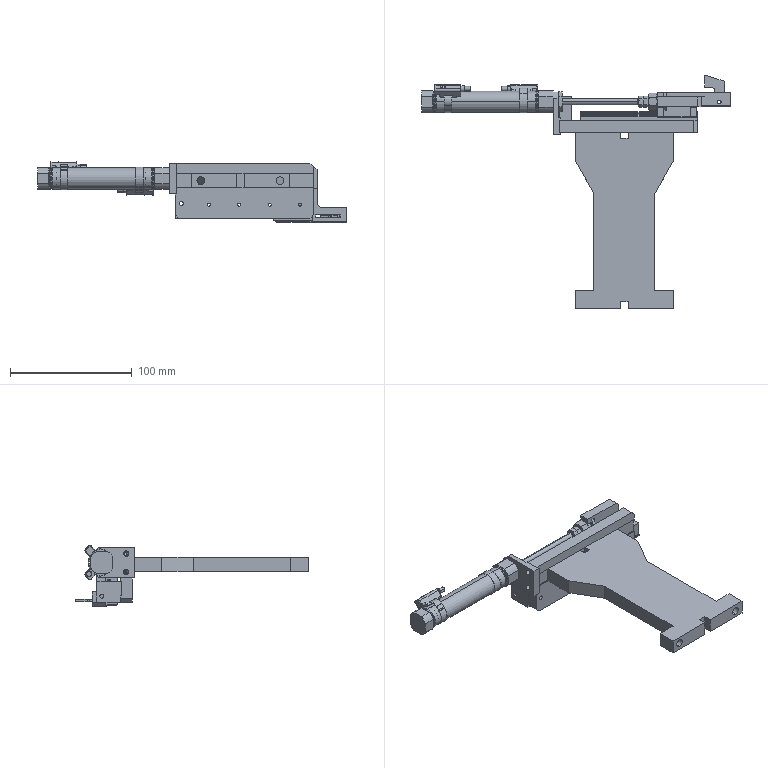Assembly | SolidWorks | mm | 16 component files | 16 solids | 740 faces | box 253.5 x 192.15 x 49.83 mm | volume 206829 mm3 | plane 324 | cylinder 258 | cone 138 | torus 16 | sphere 4 | commonest cylinder face diameters 0.5 x24 3.4 x20 10 x14 6.5 x12 5 x12 17.4 x12 3.5 x11 6 x10
Bill of materials:
17268060 | 1 | S136H FINISH:HRC50~52 degrees | Flat L-shaped plate. It has a wide square-ish section and a narrower arm running off one side. The wide section has four through holes in a rectangular pattern and an open rectangular notch on one edge. The arm has an elongated through slot and a small hole in its edge face. There are chamfered corners and shallow steps in thickness.
17268061 | 1 | SKD-11 HRC58° Electroplated | Thin flat plate with an irregular, roughly L-shaped or hook-like outline. It has one sloped edge, a rounded inside corner, a narrow tab end with chamfered corners and one through hole, and a small step notch beside the tab.
17268062 | 1 | SKD-11 HRC58° Hard Chrome Plated | Elongated rectangular bar or plate with chamfered corners. One face has a row of five larger through holes and a row of five smaller holes. A thin longitudinal groove line runs along the face, and the end views show stepped recesses on both faces.
17268063 | 1 | SKD-11 HRC58° Hard Chrome Plated | Thick rectangular plate with two chamfered corners on one end. It has two smaller through holes near one edge and one large through hole near the chamfered end. A shallow step or groove crosses one face, and the side profile is stepped.
17268064 | 1 | SKD-11 HRC58° Hard Chrome Plated | Flat plate with a symmetric dog-bone or spool outline. It has a wide rectangular head at one end, a tapered transition into a narrower central web, and a wide crossbar foot at the other end. Each end has a small central rectangular notch. Holes run into the edge faces of the foot.
17268065 | 1 | SKD-11 HRC58° Hard Chrome Plated | Rectangular block with a small step along one lower edge. It has two round holes on perpendicular faces: a larger one on one face and a smaller one on an adjacent face.
17268MGN12CZ0HM | 1 | SKD-11 HRC58° Hard Chrome Plated | Block with a C-shaped or channel cross-section. Its inner faces have longitudinal grooves with rounded profiles. The outer corners are chamfered, and stepped raised pads run along the top and bottom. Holes sit in the end face.
17268Rail-MGN12R01114HM-10_0 | 1 | SKD-11 HRC58° Hard Chrome Plated | Long straight bar of constant cross-section. A longitudinal groove with a rounded profile runs along each of two opposite faces, the corners are chamfered, and four evenly spaced round holes pass through it crosswise.
1BaseModel20210701145954 | 1 | Equivalent to S45C | Axially symmetric spool-like part with two hexagonal flanges of different lengths, joined by a narrower cylindrical neck with fillets. A central round through bore runs along the axis, and the hex corners are chamfered.
Mates:
1. concentric | 17268061-1 face at (57.5, -27.579, -8.5) dir (0, 0, -1) r 1.5 | 17268060-1 face at (57.5, -27.579, -2.5) dir (0, 0, 1) r 1.5
2. distance | 17268061-1 face at (61.5, -30.579, -8.5) dir (0, 0, 1) | 17268060-1 face at (111, -31.579, -2.5) dir (0, 0, 1)
3. parallel | 17268060-1 face at (66.5, -19.579, -14.5) dir (1, 0, 0) | 17268061-1 face at (61.5, -5.579, -10.6) dir (1, 0, 0)
4. coincident | 17268Rail-MGN12R01114HM-10_0-1 plane at (0, -43.579, 0) dir (0, 0, 1) | assembly plane at (0, 0, 0) dir (0, 0, 1)
5. coincident | 17268Rail-MGN12R01114HM-10_0-1 plane at (0, -43.579, 0) dir (1, 0, 0) | assembly plane at (0, 0, 0) dir (1, 0, 0)
6. width | 17268MGN12CZ0HM-1 face at (11.8, -37.636, -4.728) dir (0, 0.9962, 0.08707) | 17268MGN12CZ0HM-1 face at (11.8, -38.585, -5.074) dir (0, -0.9962, 0.08707) | 17268Rail-MGN12R01114HM-10_0-1 face at (56.5, -37.636, -4.728) dir (0, -0.9962, -0.08707) | 17268Rail-MGN12R01114HM-10_0-1 face at (56.5, -38.585, -5.074) dir (0, 0.9962, -0.08707)
7. width | 17268MGN12CZ0HM-1 face at (11.8, -37.885, 4.5) dir (0, 0, -1) | 17268MGN12CZ0HM-1 face at (11.8, -38.305, -4.5) dir (0, 0, 1) | 17268Rail-MGN12R01114HM-10_0-1 face at (56.5, -38.305, -4.5) dir (0, 0, -1) | 17268Rail-MGN12R01114HM-10_0-1 face at (56.5, -37.885, 4.5) dir (0, 0, 1)
8. distance | 17268MGN12CZ0HM-1 face at (38.5, -40.579, 0) dir (1, 0, 0) | 17268Rail-MGN12R01114HM-10_0-1 face at (39.5, -43.732, -6) dir (1, 0, 0)
9. distance | 17268060-1 face at (111, -31.579, -14.5) dir (0, -1, 0) | 17268MGN12CZ0HM-1 face at (33.5, -30.579, -12.9) dir (0, 1, 0)
10. distance | 17268060-1 face at (66.5, -19.579, -14.5) dir (1, 0, 0) | 17268MGN12CZ0HM-1 face at (38.5, -40.579, 0) dir (1, 0, 0)
11. distance | 17268060-1 face at (111, -31.579, -14.5) dir (0, 0, -1) | 17268MGN12CZ0HM-1 face at (33.5, -39.979, -13.5) dir (0, 0, -1)
12. distance | 17268Rail-MGN12R01114HM-10_0-1 face at (-56.5, -43.879, -2) dir (-1, 0, 0) | 17268PB16x60SU(58)+(CS1-M-2)-1/1726816PB60UBody-1 face at (-79, -27.579, 21.5) dir (1, 0, 0)
13. coincident | 17268Rail-MGN12R01114HM-10_0-1 face at (56.5, -43.579, 5.5) dir (0, -1, 0) | 17268062-1 face at (-74, -43.579, 6) dir (0, 1, 0)
14. coincident | 17268Rail-MGN12R01114HM-10_0-1 face at (39.5, -43.732, -6) dir (1, 0, 0) | 17268062-1 face at (39.5, -43.579, 0.8507) dir (1, 0, 0)
15. coincident | 17268Rail-MGN12R01114HM-10_0-1 face at (56.5, -43.079, -6) dir (0, 0, -1) | 17268062-1 face at (-74, -42.579, -6) dir (0, 0, 1)
16. coincident | 17268062-1 face at (-74, -42.579, 33.851) dir (0, 0, 1) | 17268063-1 face at (-79, -19.579, 33.851) dir (0, 0, 1)
17. distance | 17268063-1 face at (-73, -19.579, 8.851) dir (1, 0, 0) | 17268062-1 face at (-74, -43.579, 0.8507) dir (-1, 0, 0)
18. distance | 17268063-1 face at (40.5, -54.579, 0.8507) dir (0, -1, 0) | 17268062-1 face at (-74, -52.579, 33.851) dir (0, -1, 0)
19. parallel | 17268PB16x60SU(58)+(CS1-M-2)-1/1726816PB60UBody-1 face at (-90.8, -31.938, 30.5) dir (0, 0, 1) | 17268062-1 face at (-74, -42.579, 33.851) dir (0, 0, 1)
20. coincident | 17268062-1 face at (-74, -51.579, 25.851) dir (0, -1, 0) | 17268064-1 face at (39.5, -51.579, 0.8507) dir (0, 1, 0)
21. coincident | 17268062-1 face at (-74, -52.579, 25.851) dir (0, 0, -1) | 17268064-1 face at (-60.5, -197.729, 25.851) dir (0, 0, 1)
22. distance | 17268062-1 face at (39.5, -43.579, 0.8507) dir (1, 0, 0) | 17268064-1 face at (19.5, -197.729, 25.851) dir (1, 0, 0)
23. concentric | 17268PB16x60SU(58)+(CS1-M-2)-1/1726816PB60URod-1 face at (-113.36, -27.579, 21.5) dir (1, 0, 0) r 2.5 | 1BaseModel20210701145954-1 face at (-0.6, -27.579, 21.5) dir (-1, 0, 0) r 2.1
24. width | 1BaseModel20210701145954-1 face at (11.4, -27.579, 21.5) dir (-1, 0, 0) | 1BaseModel20210701145954-1 face at (14.4, -27.579, 21.5) dir (1, 0, 0) | 17268060-1 face at (14.5, -31.579, 28.8) dir (-1, 0, 0) | 17268060-1 face at (11.3, -31.579, 26.5) dir (1, 0, 0)
25. width | 1BaseModel20210701145954-1 face at (14.4, -31.043, 15.5) dir (0, 0, -1) | 1BaseModel20210701145954-1 face at (14.4, -24.115, 27.5) dir (0, 0, 1) | 17268060-1 face at (14.5, -31.579, 14.2) dir (0, 0, 1) | 17268060-1 face at (11.3, -31.579, 28.8) dir (0, 0, -1)
26. width | 17268060-1 face at (6.5, -23.579, 31.5) dir (0, 1, 0) | 17268060-1 face at (111, -31.579, -14.5) dir (0, -1, 0) | 17268PB16x60SU(58)+(CS1-M-2)-1/1726816PB60URod-1 face at (-113.36, -27.579, 21.5) dir (1, 0, 0) r 2.5
27. coincident | 1726816PB60UBody-1 axis at (-100.7, 0, 0) dir (1, 0, 0) | 1726816PB60URod-1 axis at (-178.7, 0, 0) dir (1, 0, 0)
28. angle | 1726816PB60URod-1 plane at (-97.8, 0, 0) dir (0, 0, -1) | 1726816PB60UBody-1 plane at (-19.8, 0, 0) dir (0, 0, -1)